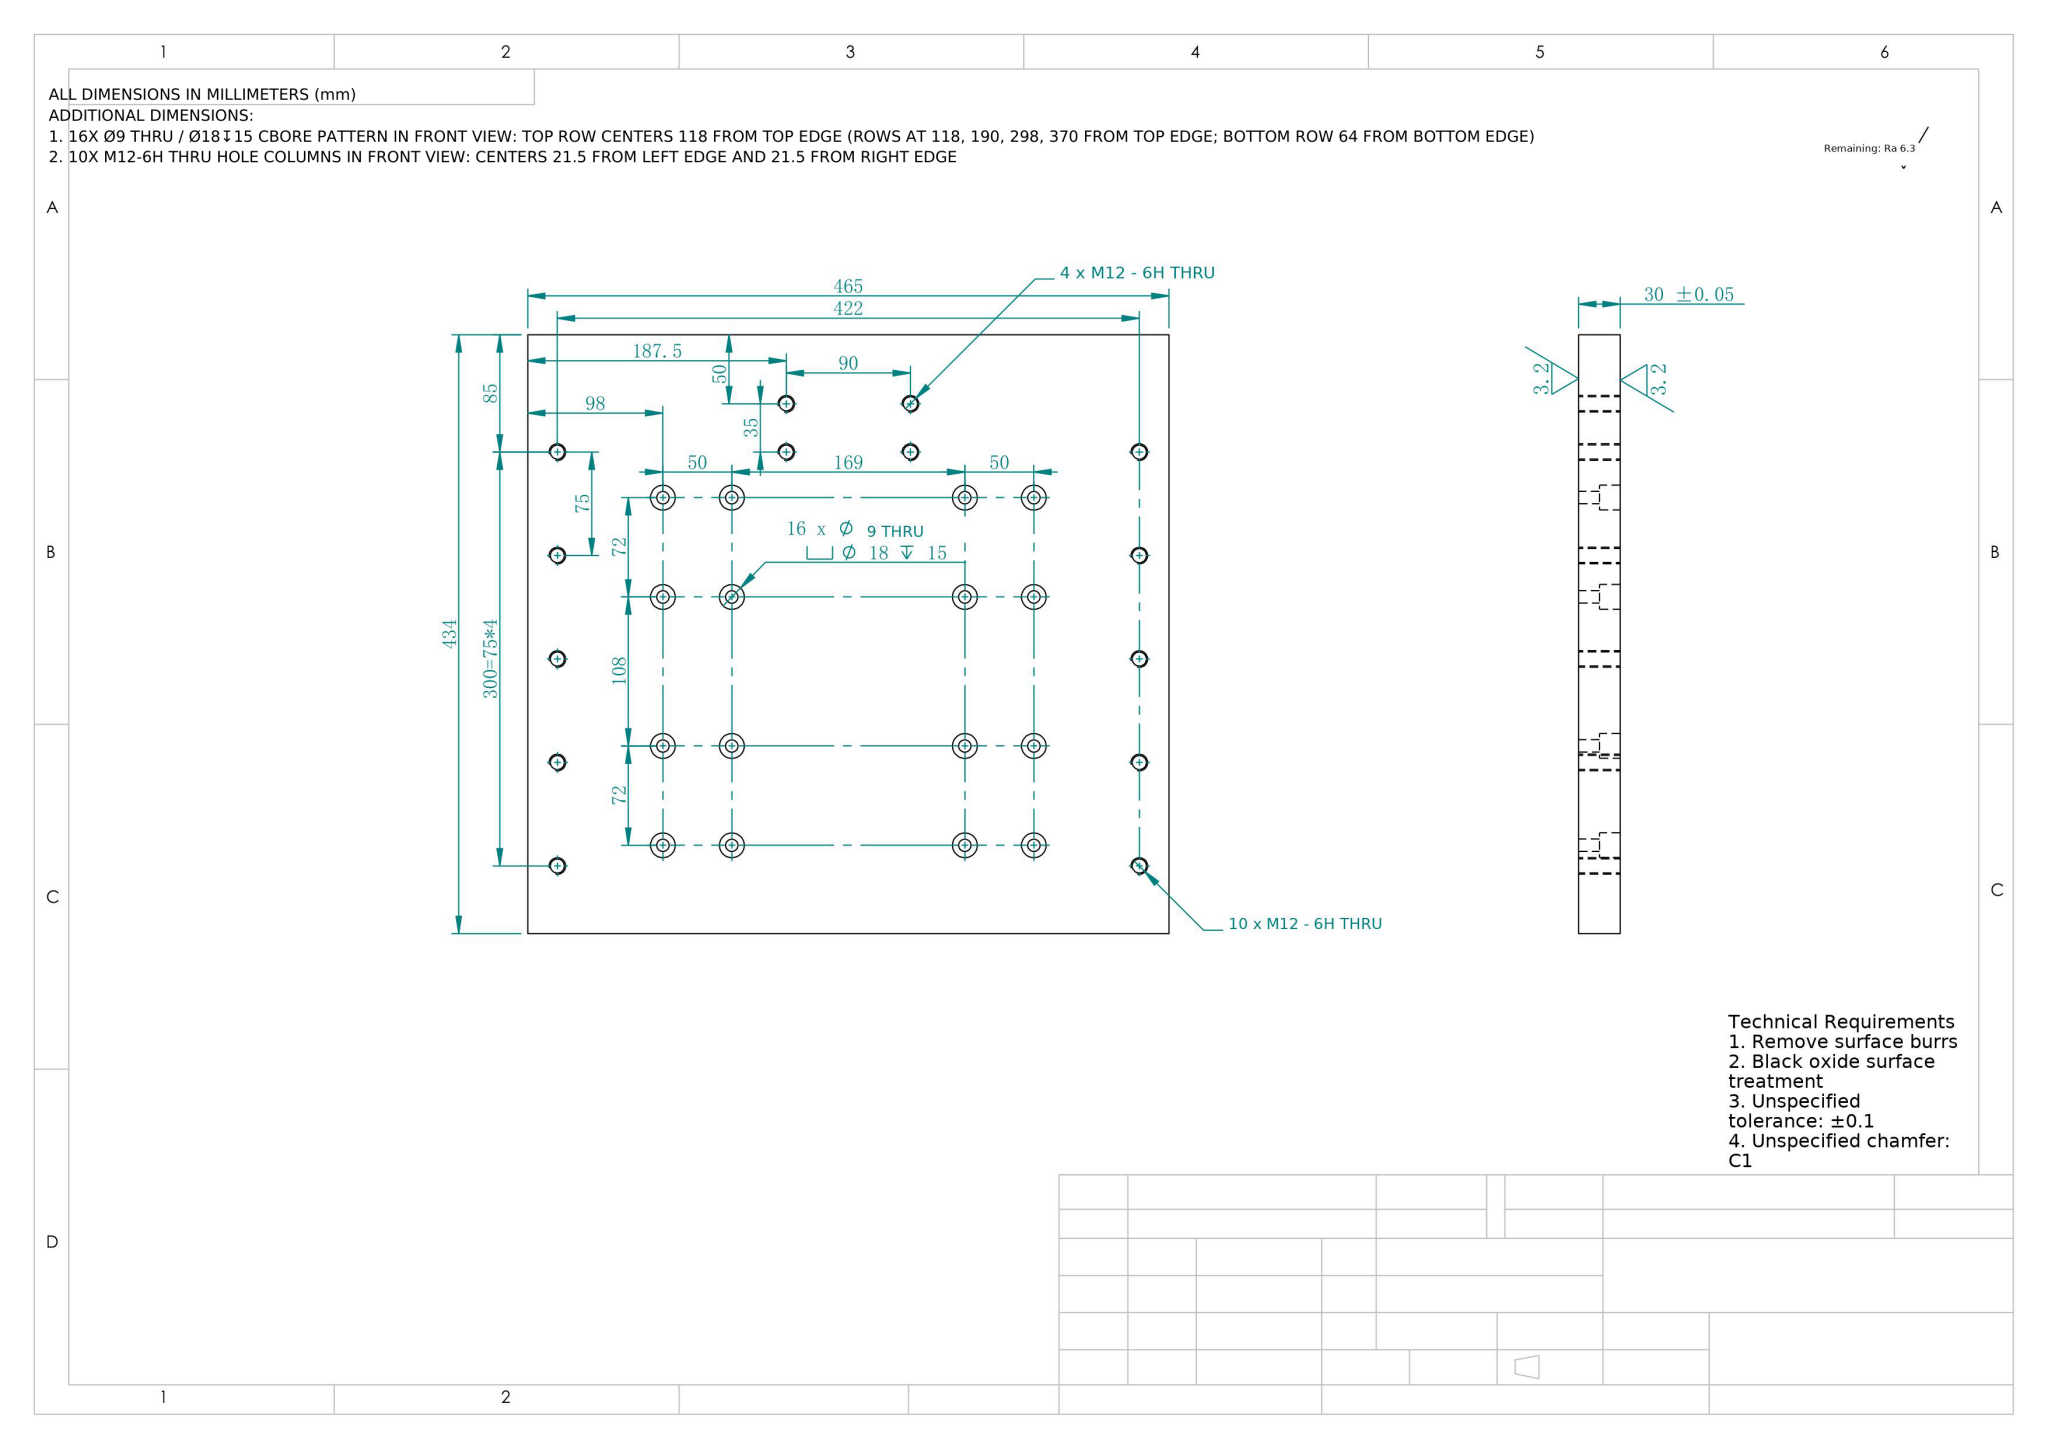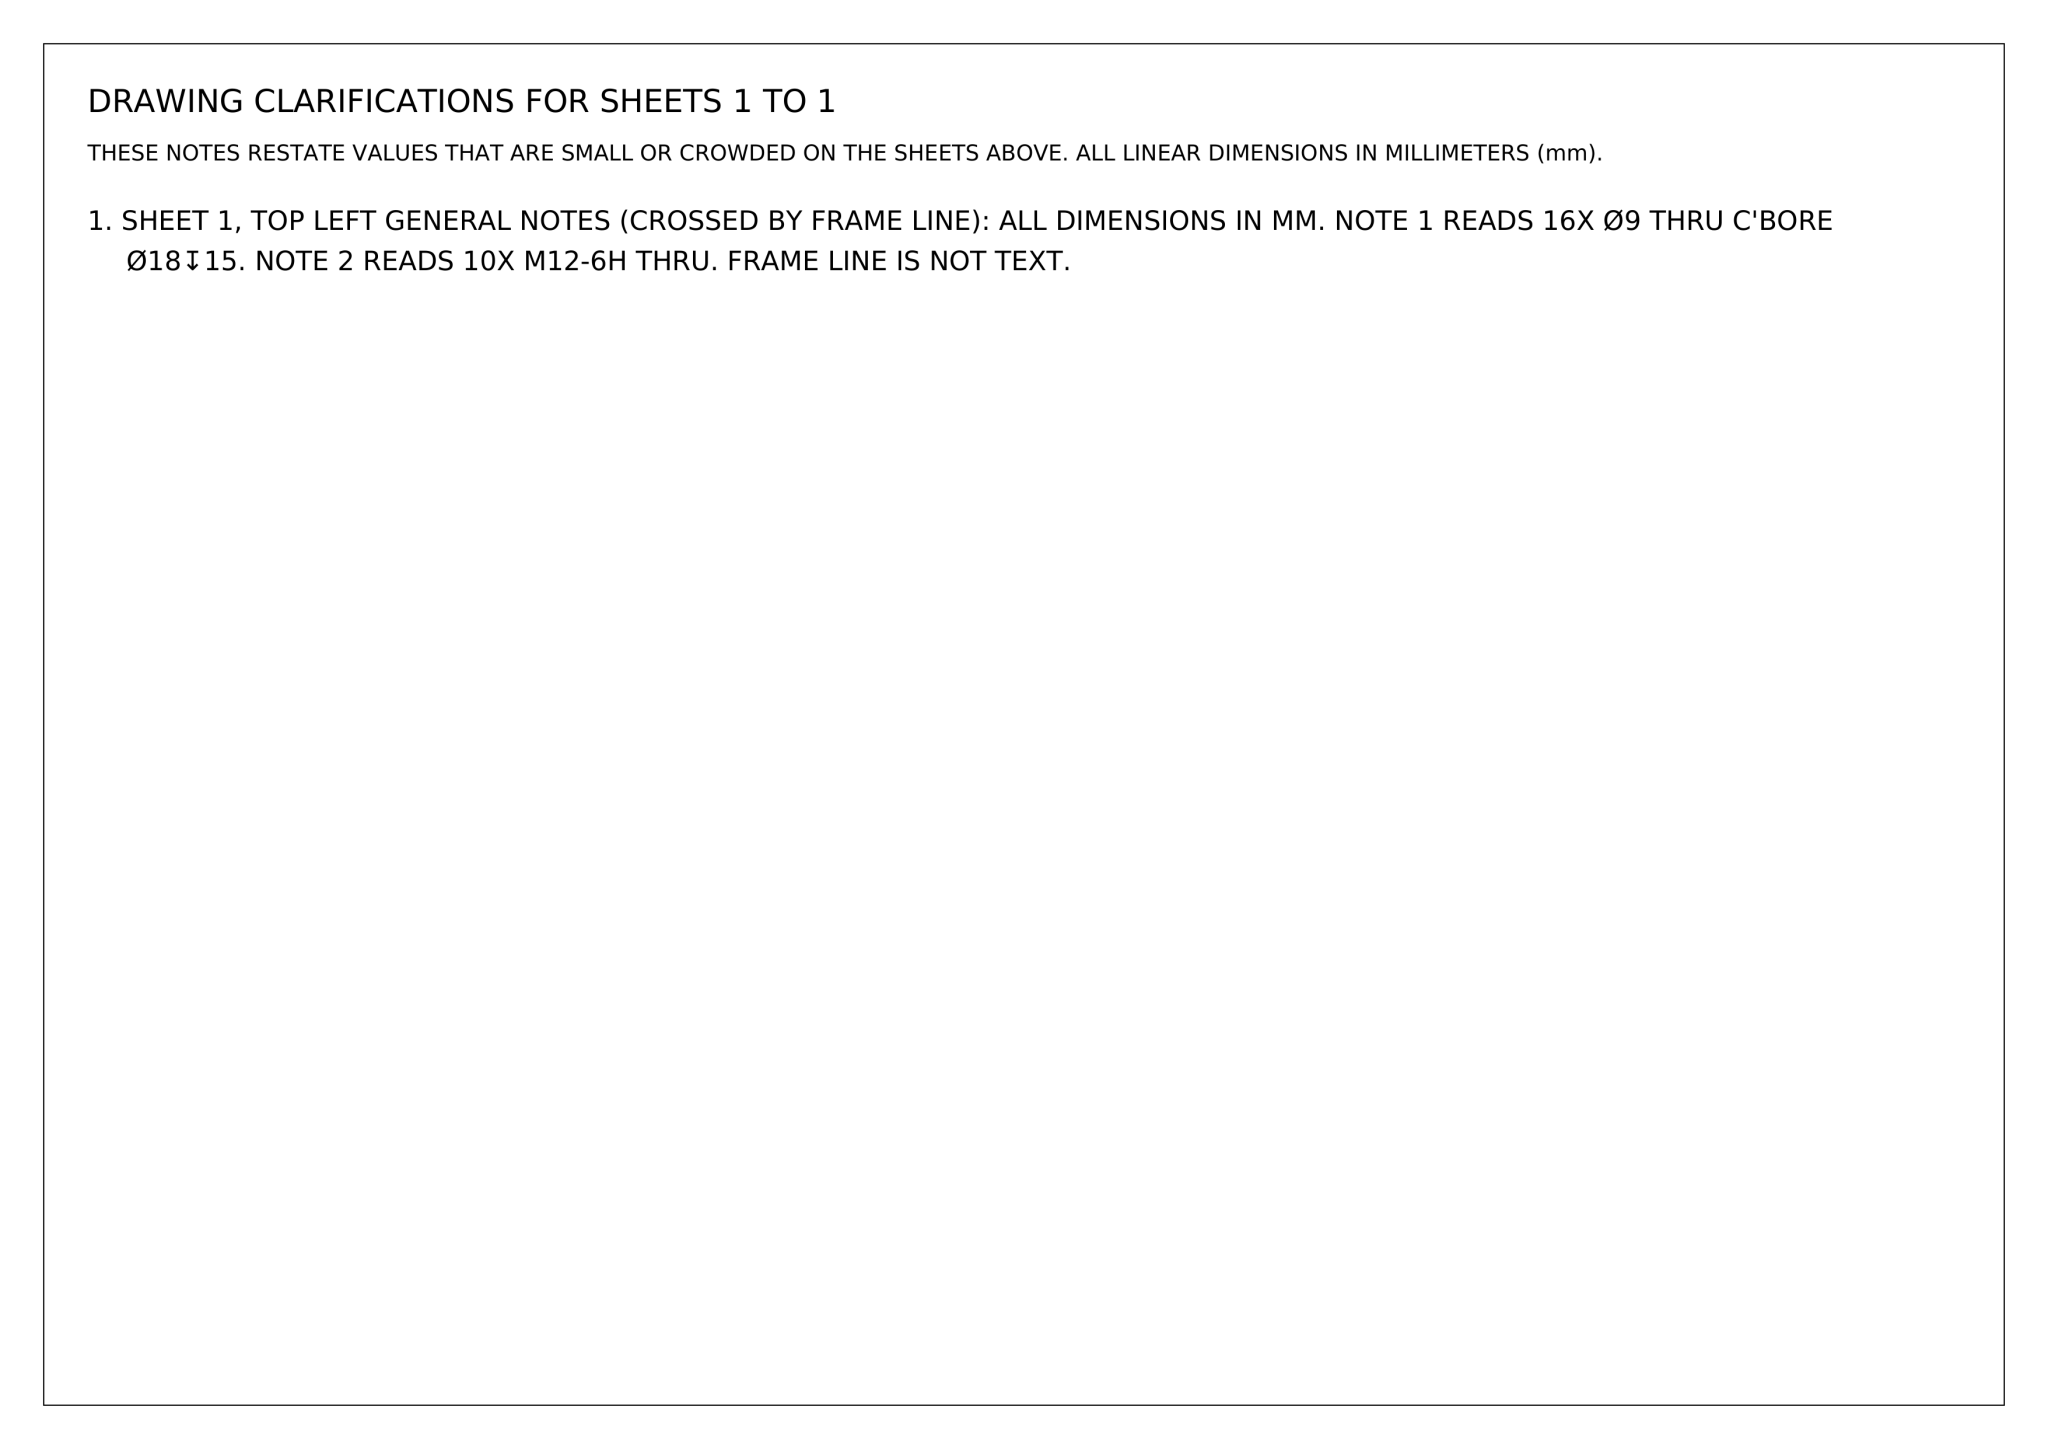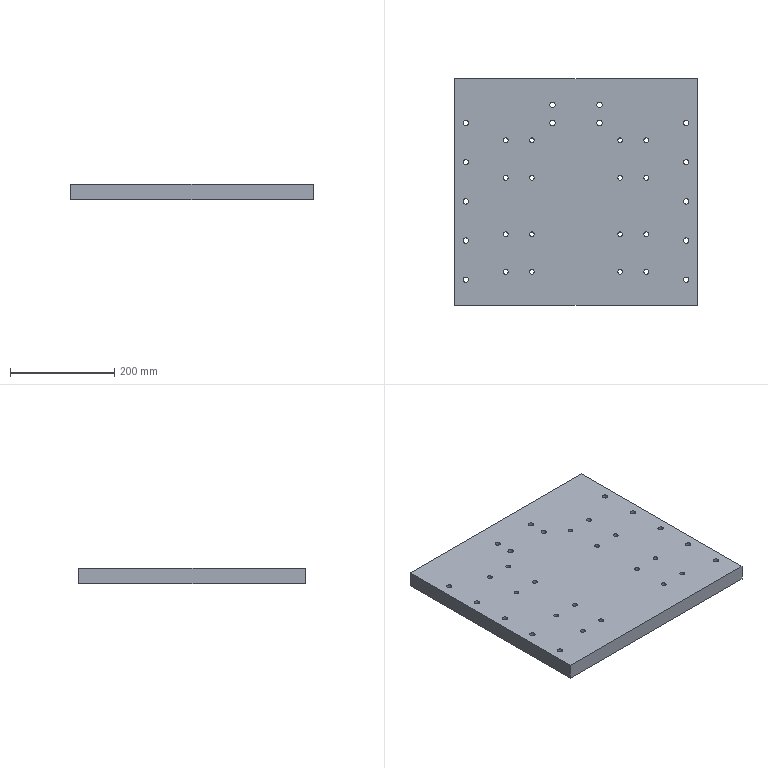Part | NX | mm | 1 solid | 114 faces | box 465 x 434 x 30 mm | volume 5943640 mm3 | cylinder 92 | plane 22 | commonest cylinder face diameters 18 x32 9 x32 10.2 x28